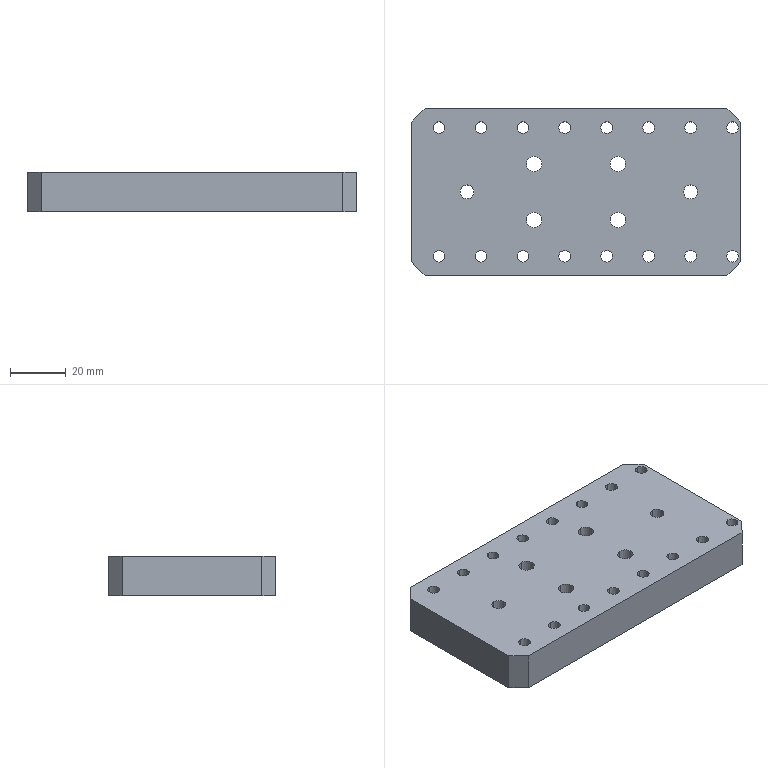Component | SolidWorks | ImagingSystem-1111-1_123456789-DL-OP20-ST12--002-1111-1 | 1 solid | 66 faces | box 118 x 60 x 14 mm | volume 92253 mm3 | cylinder 52 | plane 14 | commonest cylinder face diameters 4.2 x32 10 x8 5.5 x8 5 x4 | material AL6061 Hard Anodized Surface
build123d program:
from build123d import *

# Parameters (mm, degrees)
SKETCH1_W                                       = 250
SKETCH1_H                                       = 14
EXTRUDE1_DEPTH                                  = 60
SKETCH7_W                                       = 600
SKETCH7_H                                       = 10
CUT_EXTRUDE2_DEPTH                              = 258.48
SKETCH13_W                                      = 15
SKETCH13_H                                      = 40
BOSS_EXTRUDE1_DEPTH                             = 50
SKETCH14_W                                      = 40
SKETCH14_H                                      = 24
CUT_EXTRUDE4_DEPTH                              = 30
MOVE_FACE1_BY                                   = 10
M6_HEX_SOCKET_HEAD_CAP_SCREW_CBORE1_D           = 6.6
M6_HEX_SOCKET_HEAD_CAP_SCREW_CBORE1_CBORE_D     = 11
M6_HEX_SOCKET_HEAD_CAP_SCREW_CBORE1_CBORE_DEPTH = 6.4
SKETCH17_W                                      = 40
SKETCH17_H                                      = 16
CUT_EXTRUDE5_DEPTH                              = 30
MOVE_FACE2_BY                                   = 10
MOVE_FACE2_2_BY                                 = 10
CHAMFER1_SIZE                                   = 3
M5_TAPPED_HOLE1_AT_2_COUNT                      = 2
M5_TAPPED_HOLE1_AT_2_PITCH                      = 46
LPATTERN1_COUNT                                 = 16
LPATTERN1_PITCH                                 = 15
M5_HEX_SOCKET_HEAD_CAP_SCREW_CBORE1_D           = 5.5
M5_HEX_SOCKET_HEAD_CAP_SCREW_CBORE1_CBORE_D     = 10
M5_HEX_SOCKET_HEAD_CAP_SCREW_CBORE1_CBORE_DEPTH = 5.4
SKETCH22_W                                      = 214.509
SKETCH22_H                                      = 170.447
CUT_EXTRUDE6_DEPTH                              = 258.48
CHAMFER4_SIZE                                   = 5
SIZE_MM_DOWEL_HOLE1_D                           = 5


with BuildPart() as part:
    # Sketch1 → Extrude1 (new body)
    with BuildSketch(Plane.XY):
        with Locations((125, 7)):
            Rectangle(SKETCH1_W, SKETCH1_H)
    extrude(amount=EXTRUDE1_DEPTH)

    # Sketch7 → Cut-Extrude2 (cut, through all)
    with BuildSketch(Plane.XZ):
        with Locations((300, 5)):
            Rectangle(SKETCH7_W, SKETCH7_H)
        with Locations((300, 55)):
            Rectangle(SKETCH7_W, SKETCH7_H)
    extrude(amount=-CUT_EXTRUDE2_DEPTH, mode=Mode.SUBTRACT)

    # Sketch13 → Boss-Extrude1 (add)
    with BuildSketch(Plane(origin=(0, 14, 0), x_dir=(1, 0, 0), z_dir=(0, 1, 0))):
        with Locations((7.5, -30)):
            Rectangle(SKETCH13_W, SKETCH13_H)
    extrude(amount=BOSS_EXTRUDE1_DEPTH)

    # Sketch14 → Cut-Extrude4 (cut)
    with BuildSketch(Plane(origin=(15, 0, 0), x_dir=(0, 0, -1), z_dir=(1, 0, 0))):
        with Locations((-30, 52)):
            Rectangle(SKETCH14_W, SKETCH14_H)
    extrude(amount=-CUT_EXTRUDE4_DEPTH, mode=Mode.SUBTRACT)

    # Move Face1: a face moved inward by 10.0
    extrude(part.faces().sort_by_distance((7.5, 40, 30))[0], amount=MOVE_FACE1_BY, dir=(0, -1, 0), mode=Mode.SUBTRACT)

    # M6 Hex Socket Head Cap Screw CBORE1 (through all)
    with Locations(Plane(origin=(0, 20, 30), x_dir=(0, 0, -1), z_dir=(-1, 0, 0))):
        with Locations((0, 0)):
            CounterBoreHole(M6_HEX_SOCKET_HEAD_CAP_SCREW_CBORE1_D / 2, M6_HEX_SOCKET_HEAD_CAP_SCREW_CBORE1_CBORE_D / 2, M6_HEX_SOCKET_HEAD_CAP_SCREW_CBORE1_CBORE_DEPTH)

    # Sketch17 → Cut-Extrude5 (cut)
    with BuildSketch(Plane(origin=(15, 0, 0), x_dir=(0, 0, -1), z_dir=(1, 0, 0))):
        with Locations((-30, 22)):
            Rectangle(SKETCH17_W, SKETCH17_H)
    extrude(amount=-CUT_EXTRUDE5_DEPTH, mode=Mode.SUBTRACT)

    # Move Face2: a face moved outward by 10.0
    extrude(part.faces().sort_by_distance((125, 7, 50))[0], amount=MOVE_FACE2_BY, dir=(0, 0, 1))

    # Move Face2 2: a face moved outward by 10.0
    extrude(part.faces().sort_by_distance((125, 7, 10))[0], amount=MOVE_FACE2_2_BY, dir=(0, 0, -1))

    # Chamfer1
    chamfer1_edges = [part.edges().sort_by_distance(p)[0] for p in [
        (250, 7, 0),
        (250, 7, 60),
    ]]
    chamfer(chamfer1_edges, length=CHAMFER1_SIZE)

    # Sketch19 → M5 Tapped Hole1 (revolve, cut)
    with BuildSketch(Plane(origin=(10, 0, 53), x_dir=(0, 0, -1), z_dir=(1, 0, 0))):
        Polygon((0, 0), (0, 25.262), (2.1, 24), (2.1, 0), align=None)
    m5_tapped_hole1 = revolve(axis=Axis((10, -6.35, 53), (0, 1, 0)), mode=Mode.SUBTRACT)

    # M5 Tapped Hole1 at 2: M5 Tapped Hole1 ×2
    with Locations(*[(0, 0, -i * M5_TAPPED_HOLE1_AT_2_PITCH) for i in range(1, M5_TAPPED_HOLE1_AT_2_COUNT)]):
        add(m5_tapped_hole1, mode=Mode.SUBTRACT)

    # LPattern1: M5 Tapped Hole1 ×16
    with Locations(*[(i * LPATTERN1_PITCH, 0, 0) for i in range(1, LPATTERN1_COUNT)]):
        add(m5_tapped_hole1, mode=Mode.SUBTRACT)

    # LPattern1 copy 1 sketch → LPattern1 copy 1 (revolve, cut)
    with BuildSketch(Plane(origin=(25, 0, 7), x_dir=(0, 0, -1), z_dir=(1, 0, 0))):
        Polygon((0, 0), (0, 25.262), (2.1, 24), (2.1, 0), align=None)
    revolve(axis=Axis((25, -6.35, 7), (0, 1, 0)), mode=Mode.SUBTRACT)

    # LPattern1 copy 2 sketch → LPattern1 copy 2 (revolve, cut)
    with BuildSketch(Plane(origin=(40, 0, 7), x_dir=(0, 0, -1), z_dir=(1, 0, 0))):
        Polygon((0, 0), (0, 25.262), (2.1, 24), (2.1, 0), align=None)
    revolve(axis=Axis((40, -6.35, 7), (0, 1, 0)), mode=Mode.SUBTRACT)

    # LPattern1 copy 3 sketch → LPattern1 copy 3 (revolve, cut)
    with BuildSketch(Plane(origin=(55, 0, 7), x_dir=(0, 0, -1), z_dir=(1, 0, 0))):
        Polygon((0, 0), (0, 25.262), (2.1, 24), (2.1, 0), align=None)
    revolve(axis=Axis((55, -6.35, 7), (0, 1, 0)), mode=Mode.SUBTRACT)

    # LPattern1 copy 4 sketch → LPattern1 copy 4 (revolve, cut)
    with BuildSketch(Plane(origin=(70, 0, 7), x_dir=(0, 0, -1), z_dir=(1, 0, 0))):
        Polygon((0, 0), (0, 25.262), (2.1, 24), (2.1, 0), align=None)
    revolve(axis=Axis((70, -6.35, 7), (0, 1, 0)), mode=Mode.SUBTRACT)

    # LPattern1 copy 5 sketch → LPattern1 copy 5 (revolve, cut)
    with BuildSketch(Plane(origin=(85, 0, 7), x_dir=(0, 0, -1), z_dir=(1, 0, 0))):
        Polygon((0, 0), (0, 25.262), (2.1, 24), (2.1, 0), align=None)
    revolve(axis=Axis((85, -6.35, 7), (0, 1, 0)), mode=Mode.SUBTRACT)

    # LPattern1 copy 6 sketch → LPattern1 copy 6 (revolve, cut)
    with BuildSketch(Plane(origin=(100, 0, 7), x_dir=(0, 0, -1), z_dir=(1, 0, 0))):
        Polygon((0, 0), (0, 25.262), (2.1, 24), (2.1, 0), align=None)
    revolve(axis=Axis((100, -6.35, 7), (0, 1, 0)), mode=Mode.SUBTRACT)

    # LPattern1 copy 7 sketch → LPattern1 copy 7 (revolve, cut)
    with BuildSketch(Plane(origin=(115, 0, 7), x_dir=(0, 0, -1), z_dir=(1, 0, 0))):
        Polygon((0, 0), (0, 25.262), (2.1, 24), (2.1, 0), align=None)
    revolve(axis=Axis((115, -6.35, 7), (0, 1, 0)), mode=Mode.SUBTRACT)

    # LPattern1 copy 8 sketch → LPattern1 copy 8 (revolve, cut)
    with BuildSketch(Plane(origin=(130, 0, 7), x_dir=(0, 0, -1), z_dir=(1, 0, 0))):
        Polygon((0, 0), (0, 25.262), (2.1, 24), (2.1, 0), align=None)
    revolve(axis=Axis((130, -6.35, 7), (0, 1, 0)), mode=Mode.SUBTRACT)

    # LPattern1 copy 9 sketch → LPattern1 copy 9 (revolve, cut)
    with BuildSketch(Plane(origin=(145, 0, 7), x_dir=(0, 0, -1), z_dir=(1, 0, 0))):
        Polygon((0, 0), (0, 25.262), (2.1, 24), (2.1, 0), align=None)
    revolve(axis=Axis((145, -6.35, 7), (0, 1, 0)), mode=Mode.SUBTRACT)

    # LPattern1 copy 10 sketch → LPattern1 copy 10 (revolve, cut)
    with BuildSketch(Plane(origin=(160, 0, 7), x_dir=(0, 0, -1), z_dir=(1, 0, 0))):
        Polygon((0, 0), (0, 25.262), (2.1, 24), (2.1, 0), align=None)
    revolve(axis=Axis((160, -6.35, 7), (0, 1, 0)), mode=Mode.SUBTRACT)

    # LPattern1 copy 11 sketch → LPattern1 copy 11 (revolve, cut)
    with BuildSketch(Plane(origin=(175, 0, 7), x_dir=(0, 0, -1), z_dir=(1, 0, 0))):
        Polygon((0, 0), (0, 25.262), (2.1, 24), (2.1, 0), align=None)
    revolve(axis=Axis((175, -6.35, 7), (0, 1, 0)), mode=Mode.SUBTRACT)

    # LPattern1 copy 12 sketch → LPattern1 copy 12 (revolve, cut)
    with BuildSketch(Plane(origin=(190, 0, 7), x_dir=(0, 0, -1), z_dir=(1, 0, 0))):
        Polygon((0, 0), (0, 25.262), (2.1, 24), (2.1, 0), align=None)
    revolve(axis=Axis((190, -6.35, 7), (0, 1, 0)), mode=Mode.SUBTRACT)

    # LPattern1 copy 13 sketch → LPattern1 copy 13 (revolve, cut)
    with BuildSketch(Plane(origin=(205, 0, 7), x_dir=(0, 0, -1), z_dir=(1, 0, 0))):
        Polygon((0, 0), (0, 25.262), (2.1, 24), (2.1, 0), align=None)
    revolve(axis=Axis((205, -6.35, 7), (0, 1, 0)), mode=Mode.SUBTRACT)

    # LPattern1 copy 14 sketch → LPattern1 copy 14 (revolve, cut)
    with BuildSketch(Plane(origin=(220, 0, 7), x_dir=(0, 0, -1), z_dir=(1, 0, 0))):
        Polygon((0, 0), (0, 25.262), (2.1, 24), (2.1, 0), align=None)
    revolve(axis=Axis((220, -6.35, 7), (0, 1, 0)), mode=Mode.SUBTRACT)

    # LPattern1 copy 15 sketch → LPattern1 copy 15 (revolve, cut)
    with BuildSketch(Plane(origin=(235, 0, 7), x_dir=(0, 0, -1), z_dir=(1, 0, 0))):
        Polygon((0, 0), (0, 25.262), (2.1, 24), (2.1, 0), align=None)
    revolve(axis=Axis((235, -6.35, 7), (0, 1, 0)), mode=Mode.SUBTRACT)

    # M5 Hex Socket Head Cap Screw CBORE1 (through all)
    with Locations(Plane(origin=(0, 0, 0), x_dir=(-1, 0, 0), z_dir=(0, -1, 0))):
        with Locations((-44, -40), (-44, -20), (-74, -40), (-74, -20)):
            CounterBoreHole(M5_HEX_SOCKET_HEAD_CAP_SCREW_CBORE1_D / 2, M5_HEX_SOCKET_HEAD_CAP_SCREW_CBORE1_CBORE_D / 2, M5_HEX_SOCKET_HEAD_CAP_SCREW_CBORE1_CBORE_DEPTH)

    # Sketch22 → Cut-Extrude6 (cut, through all)
    with BuildSketch(Plane.XZ):
        with Locations((225.254, 51.325)):
            Rectangle(SKETCH22_W, SKETCH22_H)
    extrude(amount=-CUT_EXTRUDE6_DEPTH, mode=Mode.SUBTRACT)

    # Chamfer4
    chamfer4_edges = [part.edges().sort_by_distance(p)[0] for p in [
        (118, 7, 60),
        (118, 7, 0),
        (0, 7, 60),
        (0, 7, 0),
    ]]
    chamfer(chamfer4_edges, length=CHAMFER4_SIZE)

    # Size mm Dowel Hole1 (through all)
    with Locations(Plane.XZ):
        with Locations((20, 30), (100, 30)):
            Hole(SIZE_MM_DOWEL_HOLE1_D / 2)


solid = part.part

# Placed as in the assembly
solid = solid.moved(Location((-45, -25, -20), (90, 0, 0)))